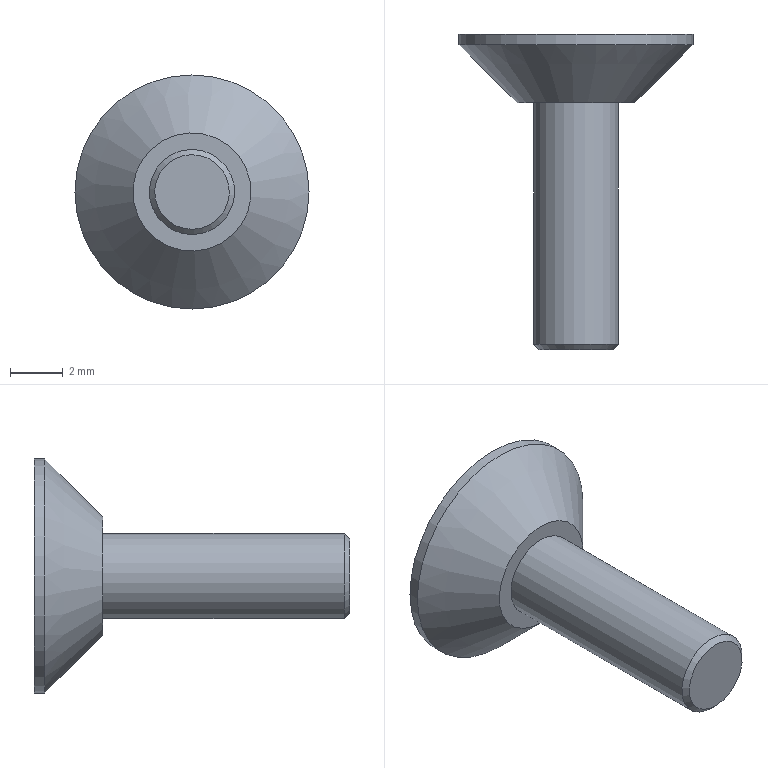Component | NX | HEX_FLAT_SCREW | 1 solid | 20 faces | volume 141 mm3 | plane 10 | cylinder 8 | cone 2 | commonest cylinder face diameters 2 x6 3.242 x1 8.907 x1